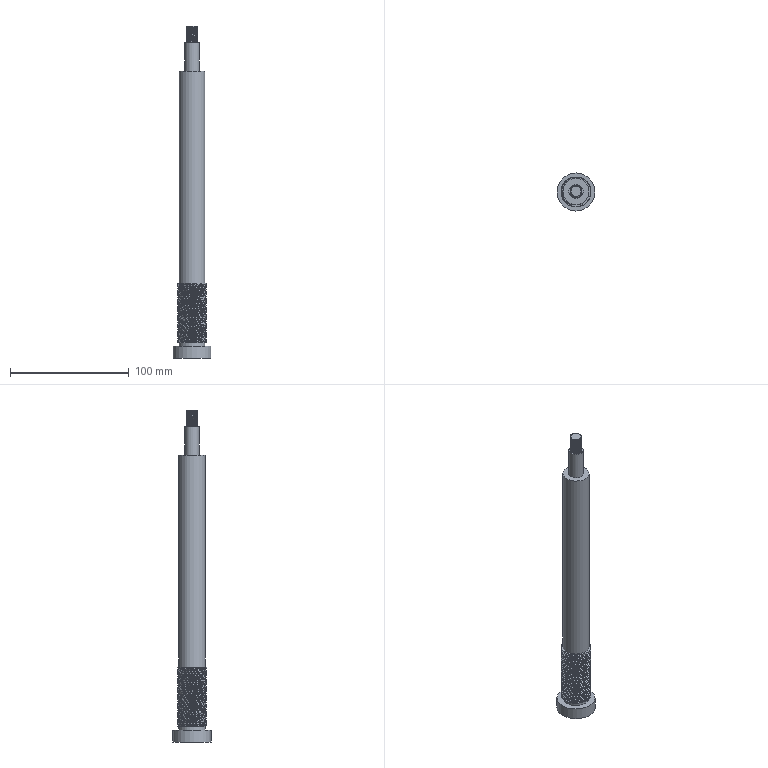Component | NX | 07__SPINDLE__2 | 1 solid | 22 faces | volume 102803 mm3 | plane 9 | cylinder 8 | spline 5 | commonest cylinder face diameters 22 x2 10 x1 12 x1 25 x1 32 x1 23.5 x1 8.5 x1